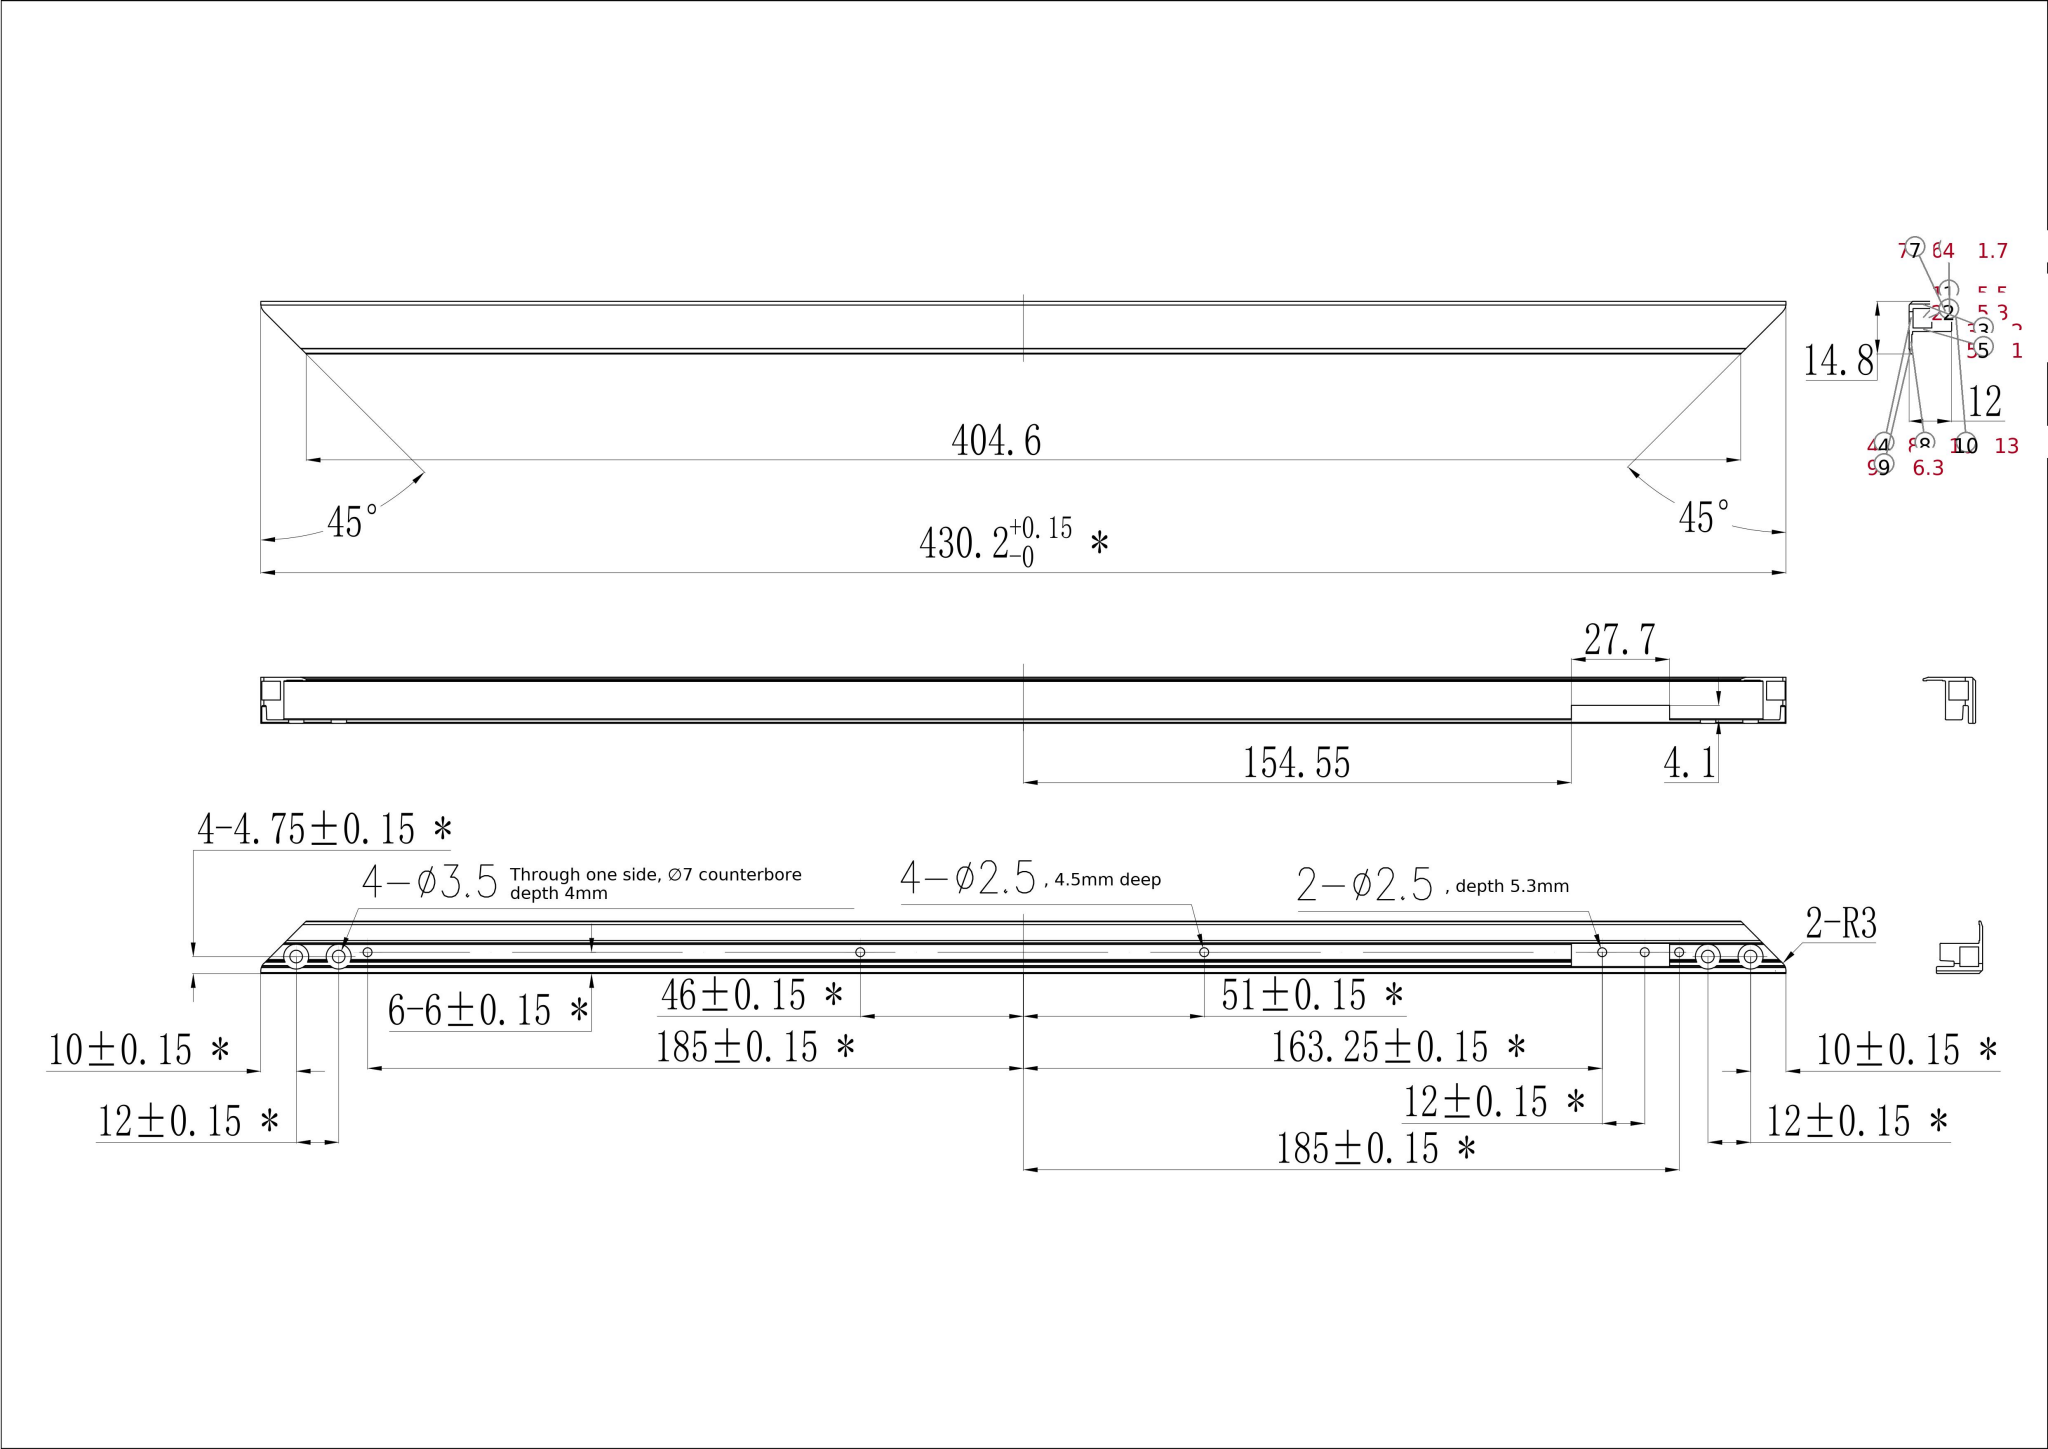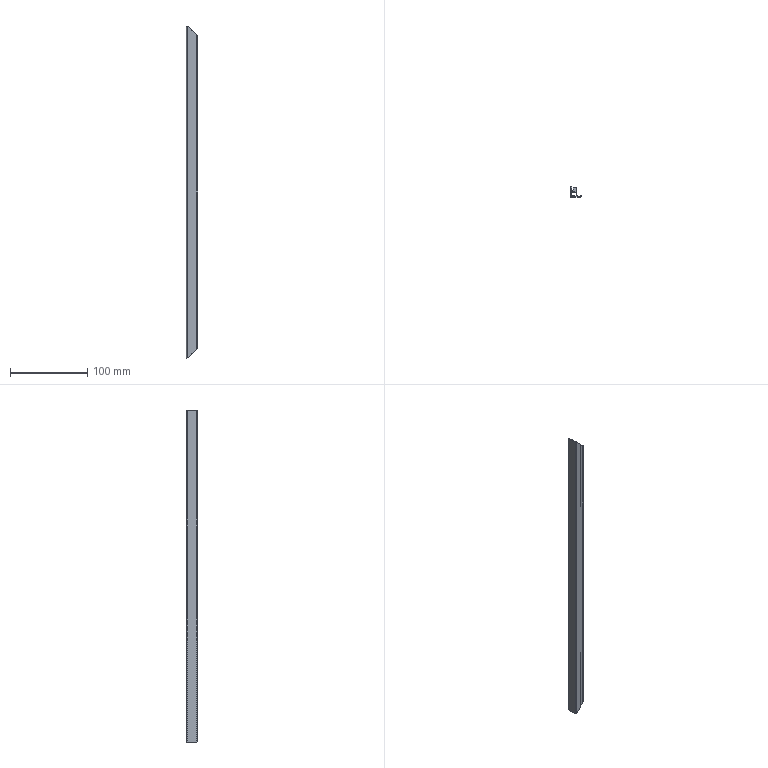Part | SolidWorks | mm | 1 solid | 116 faces | box 14.8 x 13 x 430.2 mm | volume 29742 mm3 | cylinder 68 | plane 48 | commonest cylinder face diameters 0.6 x28 7 x16 2.5 x12 3.5 x8 6 x2 0.4 x1 0.3 x1